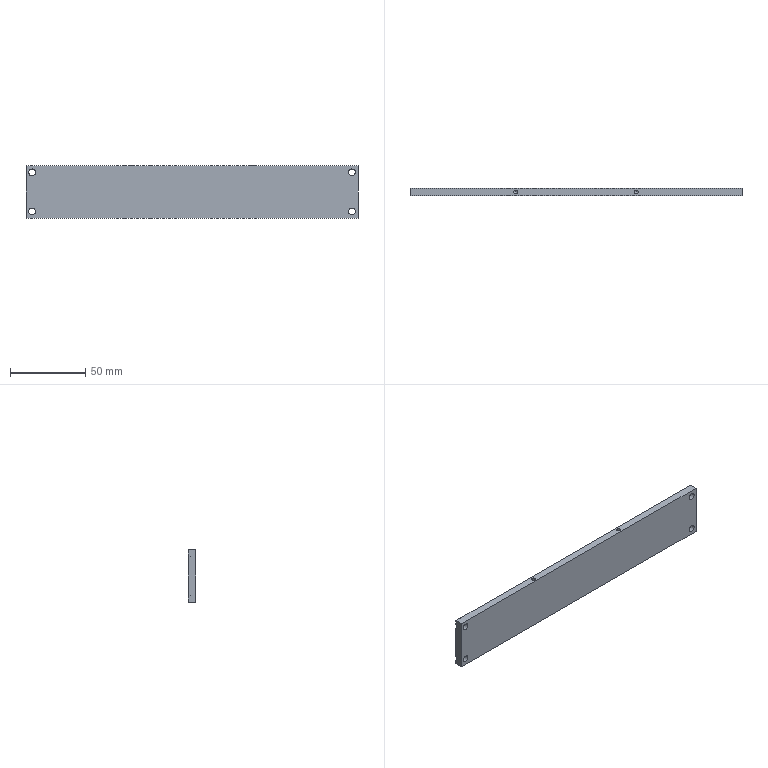CAM job | Mastercam | mm | 5 operations | part box 220 x 5 x 35
1. Contour (Ramp) | 10 - 10 平铣刀
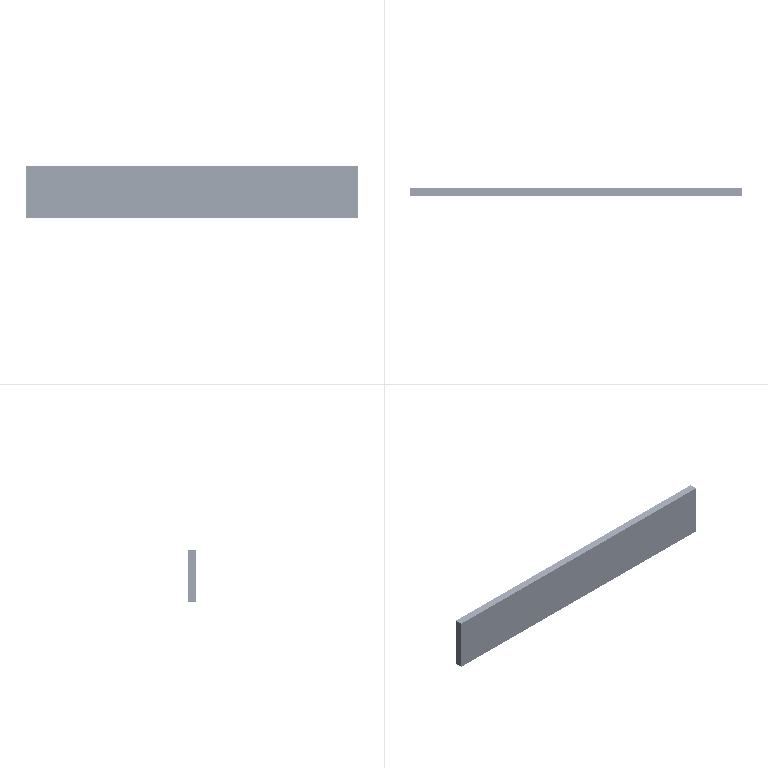2. Contour (2D) | 10 - 10 平铣刀
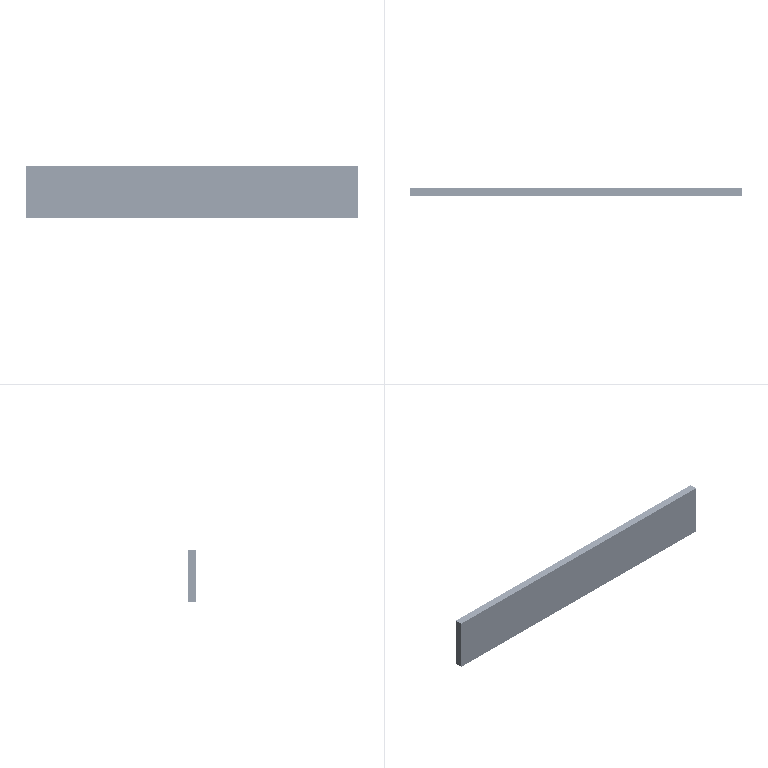3. Drill/Counterbore | 7 - 4 倒角刀
4. Contour (2D chamfer) | 7 - 4 倒角刀
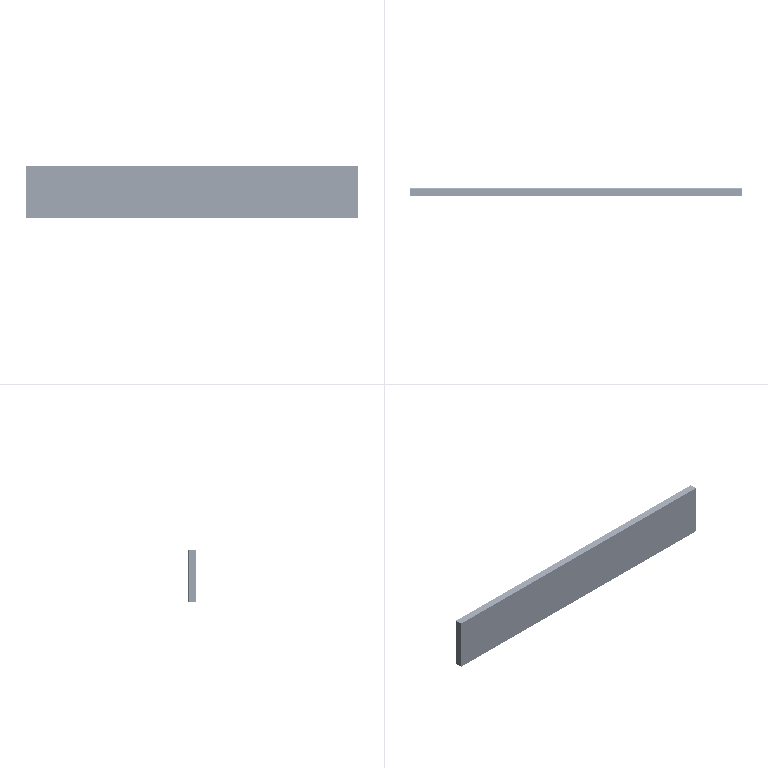5. Drill/Counterbore | 7 - 4 倒角刀